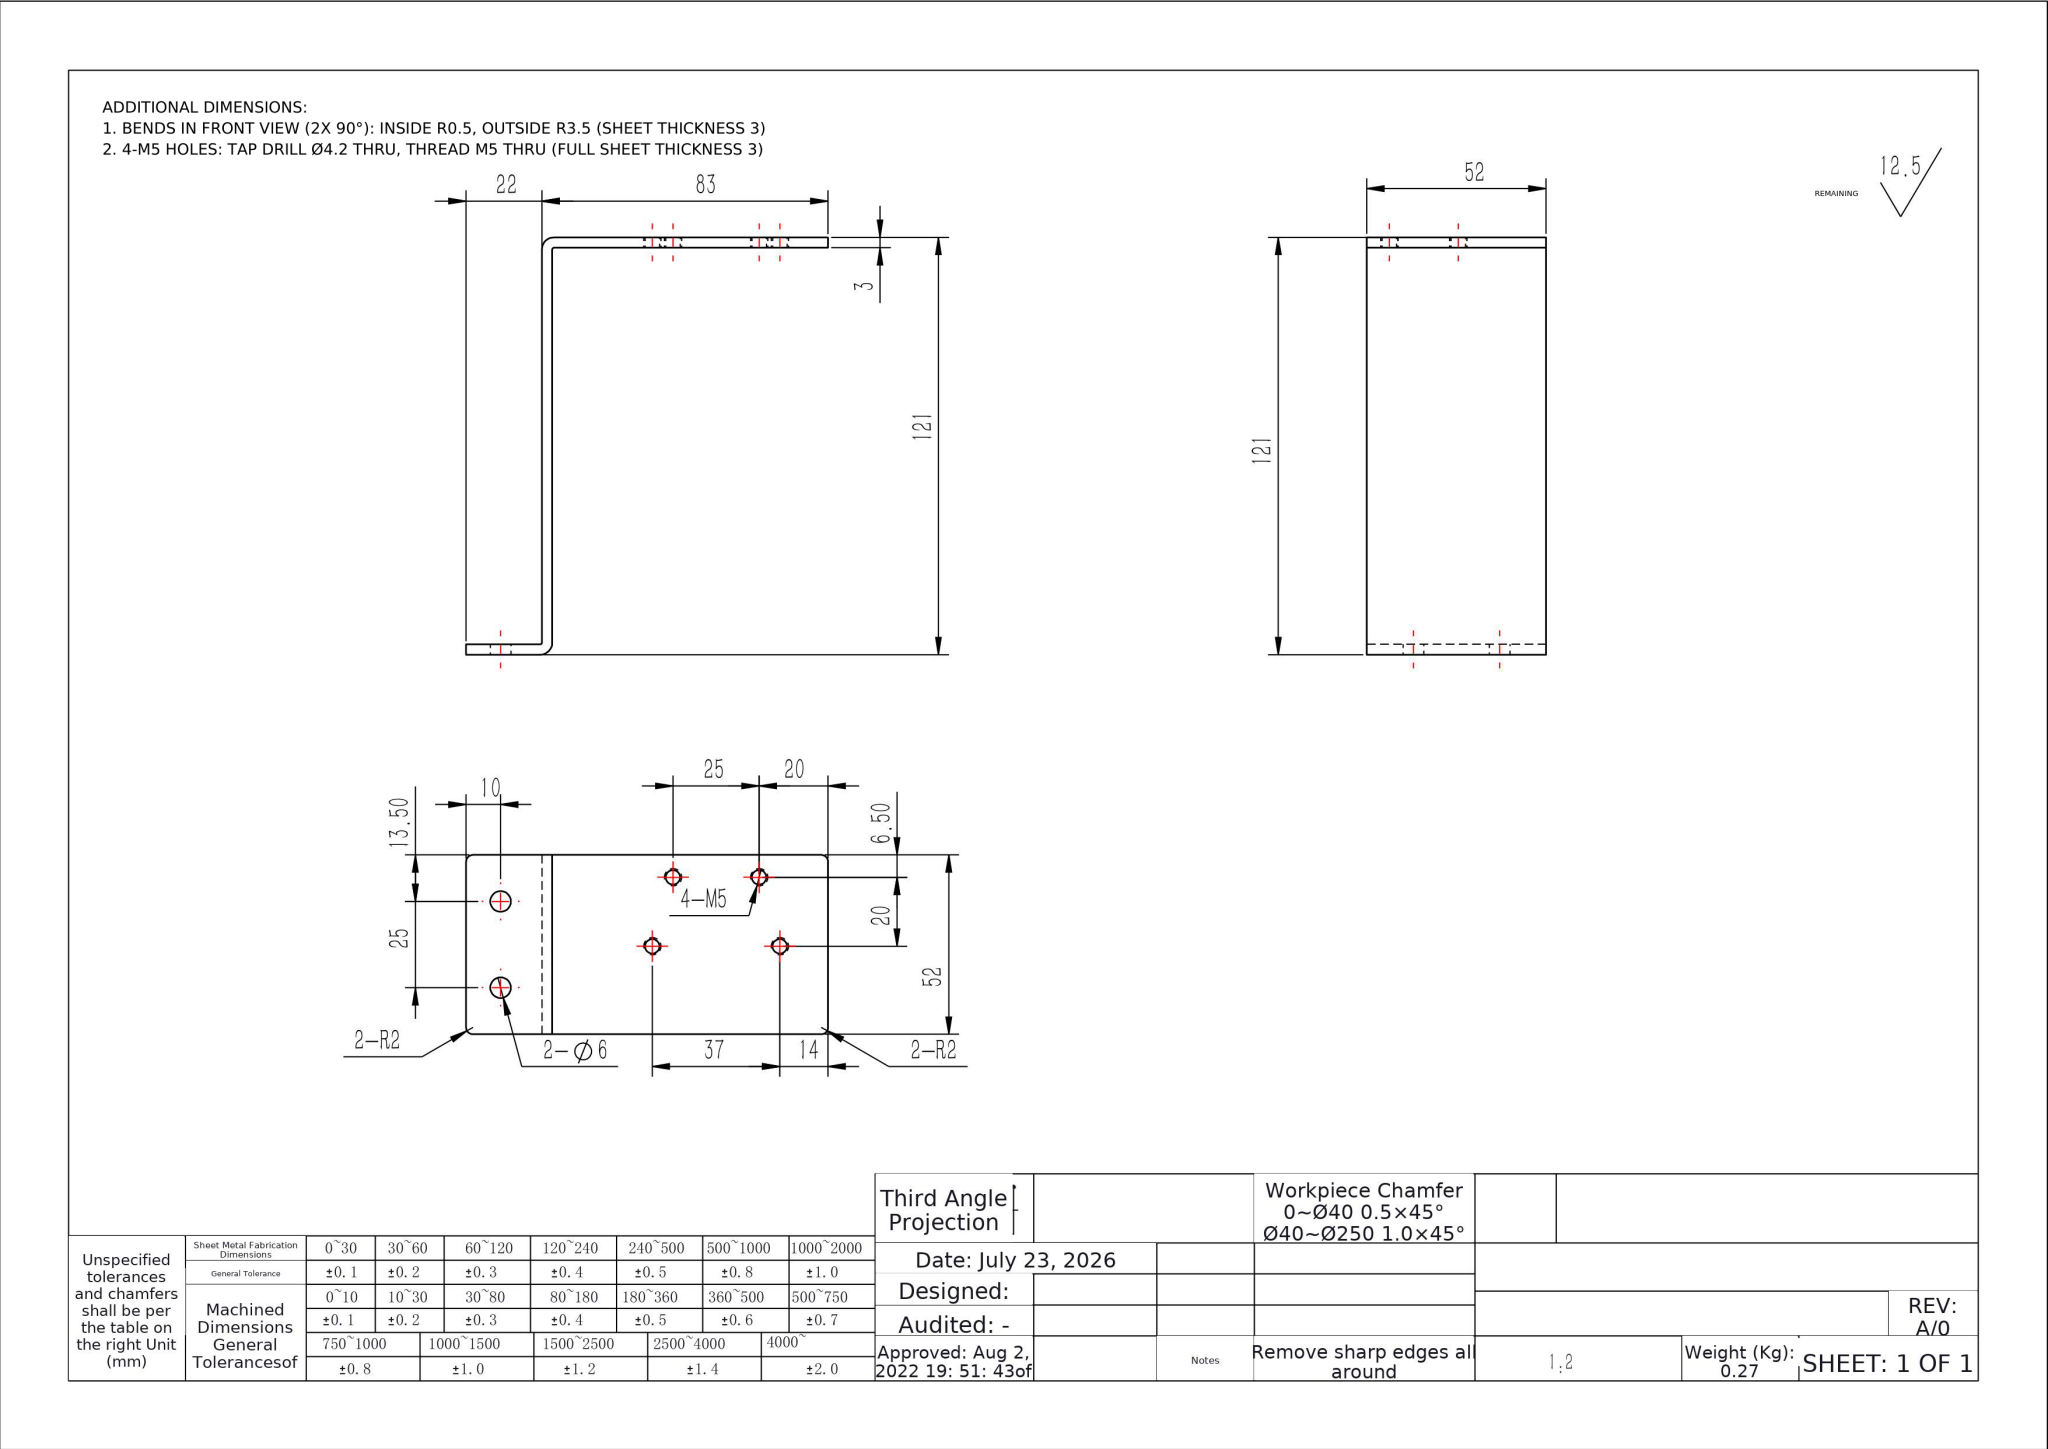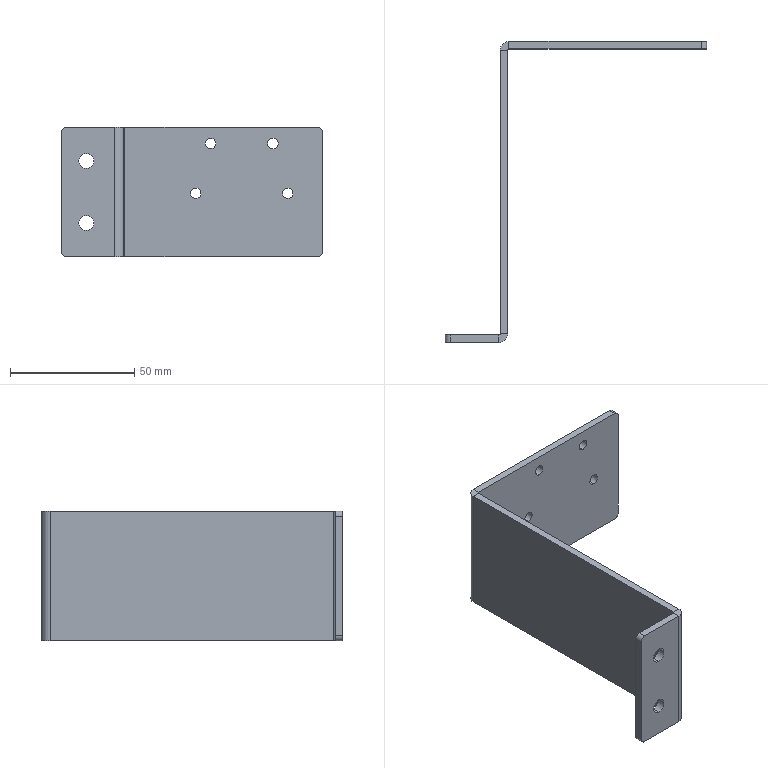Part | NX | mm | 1 solid | 38 faces | box 105 x 121 x 52 mm | volume 34174 mm3 | cylinder 20 | plane 18 | commonest cylinder face diameters 4.2 x8 6 x4 4 x4 7 x2 1 x2